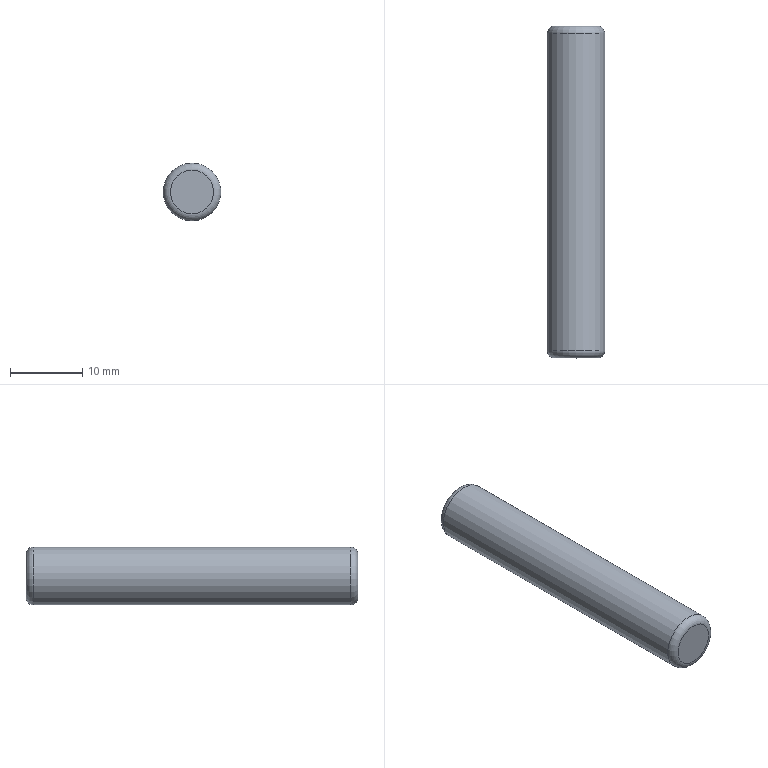Component | NX | M8 | 1 solid | 5 faces | box 8 x 46 x 8 mm | volume 2302 mm3 | plane 2 | torus 2 | cylinder 1 | commonest cylinder face diameters 8 x1
STEP:
#1=CARTESIAN_POINT('',(0.,0.,0.));
#2=DIRECTION('',(0.,0.,1.));
#3=DIRECTION('',(1.,0.,0.));
#4=AXIS2_PLACEMENT_3D('',#1,#2,#3);
#5=CARTESIAN_POINT('',(5.326,-22.,227.));
#6=VERTEX_POINT('',#5);
#7=CARTESIAN_POINT('',(5.326,-22.,224.));
#8=DIRECTION('',(0.,1.,0.));
#9=DIRECTION('',(0.,0.,1.));
#10=AXIS2_PLACEMENT_3D('',#7,#8,#9);
#11=CIRCLE('',#10,3.);
#12=CARTESIAN_POINT('',(5.326,-22.,227.));
#13=DIRECTION('',(0.,-1.,0.));
#14=DIRECTION('',(0.,0.,-1.));
#15=AXIS2_PLACEMENT_3D('',#12,#13,#14);
#16=PLANE('',#15);
#17=CARTESIAN_POINT('',(0.,0.));
#18=CARTESIAN_POINT('',(0.,5.196));
#19=CARTESIAN_POINT('',(4.5,2.598));
#20=CARTESIAN_POINT('',(9.,0.));
#21=CARTESIAN_POINT('',(4.5,-2.598));
#22=CARTESIAN_POINT('',(0.,-5.196));
#23=CARTESIAN_POINT('',(0.,0.));
#24=(BOUNDED_CURVE()B_SPLINE_CURVE(2,(#17,#18,#19,#20,#21,#22,#23),.UNSPECIFIED.,.T.,.F.)B_SPLINE_CURVE_WITH_KNOTS((1,2,2,2,2,1),(-2.094,0.,2.094,4.189,6.283,8.378),.UNSPECIFIED.)CURVE()GEOMETRIC_REPRESENTATION_ITEM()RATIONAL_B_SPLINE_CURVE((1.,0.5,1.,0.5,1.,0.5,1.))REPRESENTATION_ITEM(''));
#25=(GEOMETRIC_REPRESENTATION_CONTEXT(2)PARAMETRIC_REPRESENTATION_CONTEXT()REPRESENTATION_CONTEXT('',''));
#26=DEFINITIONAL_REPRESENTATION('',(#24),#25);
#27=PCURVE('',#16,#26);
#28=CARTESIAN_POINT('',(5.326,-21.,224.));
#29=DIRECTION('',(0.,1.,0.));
#30=DIRECTION('',(0.,0.,1.));
#31=AXIS2_PLACEMENT_3D('',#28,#29,#30);
#32=TOROIDAL_SURFACE('',#31,3.,1.);
#33=CARTESIAN_POINT('',(0.,4.712));
#34=DIRECTION('',(1.,0.));
#35=VECTOR('',#34,1.);
#36=LINE('',#33,#35);
#37=(GEOMETRIC_REPRESENTATION_CONTEXT(2)PARAMETRIC_REPRESENTATION_CONTEXT()REPRESENTATION_CONTEXT('',''));
#38=DEFINITIONAL_REPRESENTATION('',(#36),#37);
#39=PCURVE('',#32,#38);
#40=SURFACE_CURVE('',#11,(#27,#39),.PCURVE_S1.);
#41=EDGE_CURVE('',#6,#6,#40,.T.);
#42=ORIENTED_EDGE('',*,*,#41,.F.);
#43=EDGE_LOOP('',(#42));
#44=FACE_BOUND('',#43,.T.);
#45=ADVANCED_FACE('',(#44),#16,.T.);
#46=ORIENTED_EDGE('',*,*,#41,.T.);
#47=CARTESIAN_POINT('',(5.326,-21.,228.));
#48=VERTEX_POINT('',#47);
#49=CARTESIAN_POINT('',(5.326,-22.,227.));
#50=CARTESIAN_POINT('',(5.326,-22.,227.267));
#51=CARTESIAN_POINT('',(5.326,-21.915,227.528));
#52=CARTESIAN_POINT('',(5.326,-21.752,227.752));
#53=CARTESIAN_POINT('',(5.326,-21.528,227.915));
#54=CARTESIAN_POINT('',(5.326,-21.267,228.));
#55=CARTESIAN_POINT('',(5.326,-21.,228.));
#56=(BOUNDED_CURVE()B_SPLINE_CURVE(6,(#49,#50,#51,#52,#53,#54,#55),.UNSPECIFIED.,.F.,.F.)B_SPLINE_CURVE_WITH_KNOTS((7,7),(4.712,6.283),.PIECEWISE_BEZIER_KNOTS.)CURVE()GEOMETRIC_REPRESENTATION_ITEM()RATIONAL_B_SPLINE_CURVE((1.031,1.01,0.9979,0.994,0.9979,1.01,1.031))REPRESENTATION_ITEM(''));
#57=CARTESIAN_POINT('',(6.283,0.));
#58=DIRECTION('',(0.,1.));
#59=VECTOR('',#58,1.);
#60=LINE('',#57,#59);
#61=(GEOMETRIC_REPRESENTATION_CONTEXT(2)PARAMETRIC_REPRESENTATION_CONTEXT()REPRESENTATION_CONTEXT('',''));
#62=DEFINITIONAL_REPRESENTATION('',(#60),#61);
#63=PCURVE('',#32,#62);
#64=CARTESIAN_POINT('',(0.,0.));
#65=DIRECTION('',(0.,1.));
#66=VECTOR('',#65,1.);
#67=LINE('',#64,#66);
#68=(GEOMETRIC_REPRESENTATION_CONTEXT(2)PARAMETRIC_REPRESENTATION_CONTEXT()REPRESENTATION_CONTEXT('',''));
#69=DEFINITIONAL_REPRESENTATION('',(#67),#68);
#70=PCURVE('',#32,#69);
#71=SEAM_CURVE('',#56,(#63,#70),.PCURVE_S1.);
#72=EDGE_CURVE('',#6,#48,#71,.T.);
#73=ORIENTED_EDGE('',*,*,#72,.T.);
#74=CARTESIAN_POINT('',(5.326,-21.,224.));
#75=DIRECTION('',(0.,1.,0.));
#76=DIRECTION('',(0.,0.,1.));
#77=AXIS2_PLACEMENT_3D('',#74,#75,#76);
#78=CIRCLE('',#77,4.);
#79=CARTESIAN_POINT('',(0.,6.283));
#80=DIRECTION('',(1.,0.));
#81=VECTOR('',#80,1.);
#82=LINE('',#79,#81);
#83=(GEOMETRIC_REPRESENTATION_CONTEXT(2)PARAMETRIC_REPRESENTATION_CONTEXT()REPRESENTATION_CONTEXT('',''));
#84=DEFINITIONAL_REPRESENTATION('',(#82),#83);
#85=PCURVE('',#32,#84);
#86=CARTESIAN_POINT('',(5.326,63.399,224.));
#87=DIRECTION('',(0.,1.,0.));
#88=DIRECTION('',(0.,0.,1.));
#89=AXIS2_PLACEMENT_3D('',#86,#87,#88);
#90=CYLINDRICAL_SURFACE('',#89,4.);
#91=CARTESIAN_POINT('',(0.,-84.399));
#92=DIRECTION('',(1.,0.));
#93=VECTOR('',#92,1.);
#94=LINE('',#91,#93);
#95=(GEOMETRIC_REPRESENTATION_CONTEXT(2)PARAMETRIC_REPRESENTATION_CONTEXT()REPRESENTATION_CONTEXT('',''));
#96=DEFINITIONAL_REPRESENTATION('',(#94),#95);
#97=PCURVE('',#90,#96);
#98=SURFACE_CURVE('',#78,(#85,#97),.PCURVE_S1.);
#99=EDGE_CURVE('',#48,#48,#98,.T.);
#100=ORIENTED_EDGE('',*,*,#99,.F.);
#101=ORIENTED_EDGE('',*,*,#72,.F.);
#102=EDGE_LOOP('',(#46,#73,#100,#101));
#103=FACE_BOUND('',#102,.T.);
#104=ADVANCED_FACE('',(#103),#32,.T.);
#105=ORIENTED_EDGE('',*,*,#99,.T.);
#106=CARTESIAN_POINT('',(5.326,23.,228.));
#107=VERTEX_POINT('',#106);
#108=CARTESIAN_POINT('',(5.326,-21.,228.));
#109=CARTESIAN_POINT('',(5.326,23.,228.));
#110=B_SPLINE_CURVE_WITH_KNOTS('',1,(#108,#109),.UNSPECIFIED.,.F.,.F.,(2,2),(-84.399,-40.399),.PIECEWISE_BEZIER_KNOTS.);
#111=CARTESIAN_POINT('',(6.283,0.));
#112=DIRECTION('',(0.,1.));
#113=VECTOR('',#112,1.);
#114=LINE('',#111,#113);
#115=(GEOMETRIC_REPRESENTATION_CONTEXT(2)PARAMETRIC_REPRESENTATION_CONTEXT()REPRESENTATION_CONTEXT('',''));
#116=DEFINITIONAL_REPRESENTATION('',(#114),#115);
#117=PCURVE('',#90,#116);
#118=CARTESIAN_POINT('',(0.,0.));
#119=DIRECTION('',(0.,1.));
#120=VECTOR('',#119,1.);
#121=LINE('',#118,#120);
#122=(GEOMETRIC_REPRESENTATION_CONTEXT(2)PARAMETRIC_REPRESENTATION_CONTEXT()REPRESENTATION_CONTEXT('',''));
#123=DEFINITIONAL_REPRESENTATION('',(#121),#122);
#124=PCURVE('',#90,#123);
#125=SEAM_CURVE('',#110,(#117,#124),.PCURVE_S1.);
#126=EDGE_CURVE('',#48,#107,#125,.T.);
#127=ORIENTED_EDGE('',*,*,#126,.T.);
#128=CARTESIAN_POINT('',(5.326,23.,224.));
#129=DIRECTION('',(0.,1.,0.));
#130=DIRECTION('',(0.,0.,1.));
#131=AXIS2_PLACEMENT_3D('',#128,#129,#130);
#132=CIRCLE('',#131,4.);
#133=CARTESIAN_POINT('',(0.,-40.399));
#134=DIRECTION('',(1.,0.));
#135=VECTOR('',#134,1.);
#136=LINE('',#133,#135);
#137=(GEOMETRIC_REPRESENTATION_CONTEXT(2)PARAMETRIC_REPRESENTATION_CONTEXT()REPRESENTATION_CONTEXT('',''));
#138=DEFINITIONAL_REPRESENTATION('',(#136),#137);
#139=PCURVE('',#90,#138);
#140=CARTESIAN_POINT('',(5.326,23.,224.));
#141=DIRECTION('',(0.,1.,0.));
#142=DIRECTION('',(0.,0.,1.));
#143=AXIS2_PLACEMENT_3D('',#140,#141,#142);
#144=TOROIDAL_SURFACE('',#143,3.,1.);
#145=CARTESIAN_POINT('',(0.,6.283));
#146=DIRECTION('',(1.,0.));
#147=VECTOR('',#146,1.);
#148=LINE('',#145,#147);
#149=(GEOMETRIC_REPRESENTATION_CONTEXT(2)PARAMETRIC_REPRESENTATION_CONTEXT()REPRESENTATION_CONTEXT('',''));
#150=DEFINITIONAL_REPRESENTATION('',(#148),#149);
#151=PCURVE('',#144,#150);
#152=SURFACE_CURVE('',#132,(#139,#151),.PCURVE_S1.);
#153=EDGE_CURVE('',#107,#107,#152,.T.);
#154=ORIENTED_EDGE('',*,*,#153,.F.);
#155=ORIENTED_EDGE('',*,*,#126,.F.);
#156=EDGE_LOOP('',(#105,#127,#154,#155));
#157=FACE_BOUND('',#156,.T.);
#158=ADVANCED_FACE('',(#157),#90,.T.);
#159=ORIENTED_EDGE('',*,*,#153,.T.);
#160=CARTESIAN_POINT('',(5.326,24.,227.));
#161=VERTEX_POINT('',#160);
#162=CARTESIAN_POINT('',(5.326,23.,228.));
#163=CARTESIAN_POINT('',(5.326,23.267,228.));
#164=CARTESIAN_POINT('',(5.326,23.528,227.915));
#165=CARTESIAN_POINT('',(5.326,23.752,227.752));
#166=CARTESIAN_POINT('',(5.326,23.915,227.528));
#167=CARTESIAN_POINT('',(5.326,24.,227.267));
#168=CARTESIAN_POINT('',(5.326,24.,227.));
#169=(BOUNDED_CURVE()B_SPLINE_CURVE(6,(#162,#163,#164,#165,#166,#167,#168),.UNSPECIFIED.,.F.,.F.)B_SPLINE_CURVE_WITH_KNOTS((7,7),(0.,1.571),.PIECEWISE_BEZIER_KNOTS.)CURVE()GEOMETRIC_REPRESENTATION_ITEM()RATIONAL_B_SPLINE_CURVE((1.031,1.01,0.9979,0.994,0.9979,1.01,1.031))REPRESENTATION_ITEM(''));
#170=CARTESIAN_POINT('',(6.283,6.283));
#171=DIRECTION('',(0.,1.));
#172=VECTOR('',#171,1.);
#173=LINE('',#170,#172);
#174=(GEOMETRIC_REPRESENTATION_CONTEXT(2)PARAMETRIC_REPRESENTATION_CONTEXT()REPRESENTATION_CONTEXT('',''));
#175=DEFINITIONAL_REPRESENTATION('',(#173),#174);
#176=PCURVE('',#144,#175);
#177=CARTESIAN_POINT('',(0.,6.283));
#178=DIRECTION('',(0.,1.));
#179=VECTOR('',#178,1.);
#180=LINE('',#177,#179);
#181=(GEOMETRIC_REPRESENTATION_CONTEXT(2)PARAMETRIC_REPRESENTATION_CONTEXT()REPRESENTATION_CONTEXT('',''));
#182=DEFINITIONAL_REPRESENTATION('',(#180),#181);
#183=PCURVE('',#144,#182);
#184=SEAM_CURVE('',#169,(#176,#183),.PCURVE_S1.);
#185=EDGE_CURVE('',#107,#161,#184,.T.);
#186=ORIENTED_EDGE('',*,*,#185,.T.);
#187=CARTESIAN_POINT('',(5.326,24.,224.));
#188=DIRECTION('',(0.,1.,0.));
#189=DIRECTION('',(0.,0.,1.));
#190=AXIS2_PLACEMENT_3D('',#187,#188,#189);
#191=CIRCLE('',#190,3.);
#192=CARTESIAN_POINT('',(0.,7.854));
#193=DIRECTION('',(1.,0.));
#194=VECTOR('',#193,1.);
#195=LINE('',#192,#194);
#196=(GEOMETRIC_REPRESENTATION_CONTEXT(2)PARAMETRIC_REPRESENTATION_CONTEXT()REPRESENTATION_CONTEXT('',''));
#197=DEFINITIONAL_REPRESENTATION('',(#195),#196);
#198=PCURVE('',#144,#197);
#199=CARTESIAN_POINT('',(5.326,24.,224.));
#200=DIRECTION('',(0.,1.,0.));
#201=DIRECTION('',(0.,0.,1.));
#202=AXIS2_PLACEMENT_3D('',#199,#200,#201);
#203=PLANE('',#202);
#204=CARTESIAN_POINT('',(0.,0.));
#205=DIRECTION('',(1.,0.));
#206=AXIS2_PLACEMENT_2D('',#204,#205);
#207=CIRCLE('',#206,3.);
#208=(GEOMETRIC_REPRESENTATION_CONTEXT(2)PARAMETRIC_REPRESENTATION_CONTEXT()REPRESENTATION_CONTEXT('',''));
#209=DEFINITIONAL_REPRESENTATION('',(#207),#208);
#210=PCURVE('',#203,#209);
#211=SURFACE_CURVE('',#191,(#198,#210),.PCURVE_S1.);
#212=EDGE_CURVE('',#161,#161,#211,.T.);
#213=ORIENTED_EDGE('',*,*,#212,.F.);
#214=ORIENTED_EDGE('',*,*,#185,.F.);
#215=EDGE_LOOP('',(#159,#186,#213,#214));
#216=FACE_BOUND('',#215,.T.);
#217=ADVANCED_FACE('',(#216),#144,.T.);
#218=ORIENTED_EDGE('',*,*,#212,.T.);
#219=EDGE_LOOP('',(#218));
#220=FACE_BOUND('',#219,.T.);
#221=ADVANCED_FACE('',(#220),#203,.T.);
#222=CLOSED_SHELL('',(#45,#104,#158,#217,#221));
#223=MANIFOLD_SOLID_BREP('',#222);
#224=(LENGTH_UNIT()NAMED_UNIT(*)SI_UNIT(.MILLI.,.METRE.));
#225=UNCERTAINTY_MEASURE_WITH_UNIT(LENGTH_MEASURE(0.00001),#224,'','');
#226=(NAMED_UNIT(*)PLANE_ANGLE_UNIT()SI_UNIT($,.RADIAN.));
#227=(NAMED_UNIT(*)SI_UNIT($,.STERADIAN.)SOLID_ANGLE_UNIT());
#228=(GEOMETRIC_REPRESENTATION_CONTEXT(3)GLOBAL_UNCERTAINTY_ASSIGNED_CONTEXT((#225))GLOBAL_UNIT_ASSIGNED_CONTEXT((#224,#226,#227))REPRESENTATION_CONTEXT('',''));
#229=ADVANCED_BREP_SHAPE_REPRESENTATION('',(#4,#223),#228);